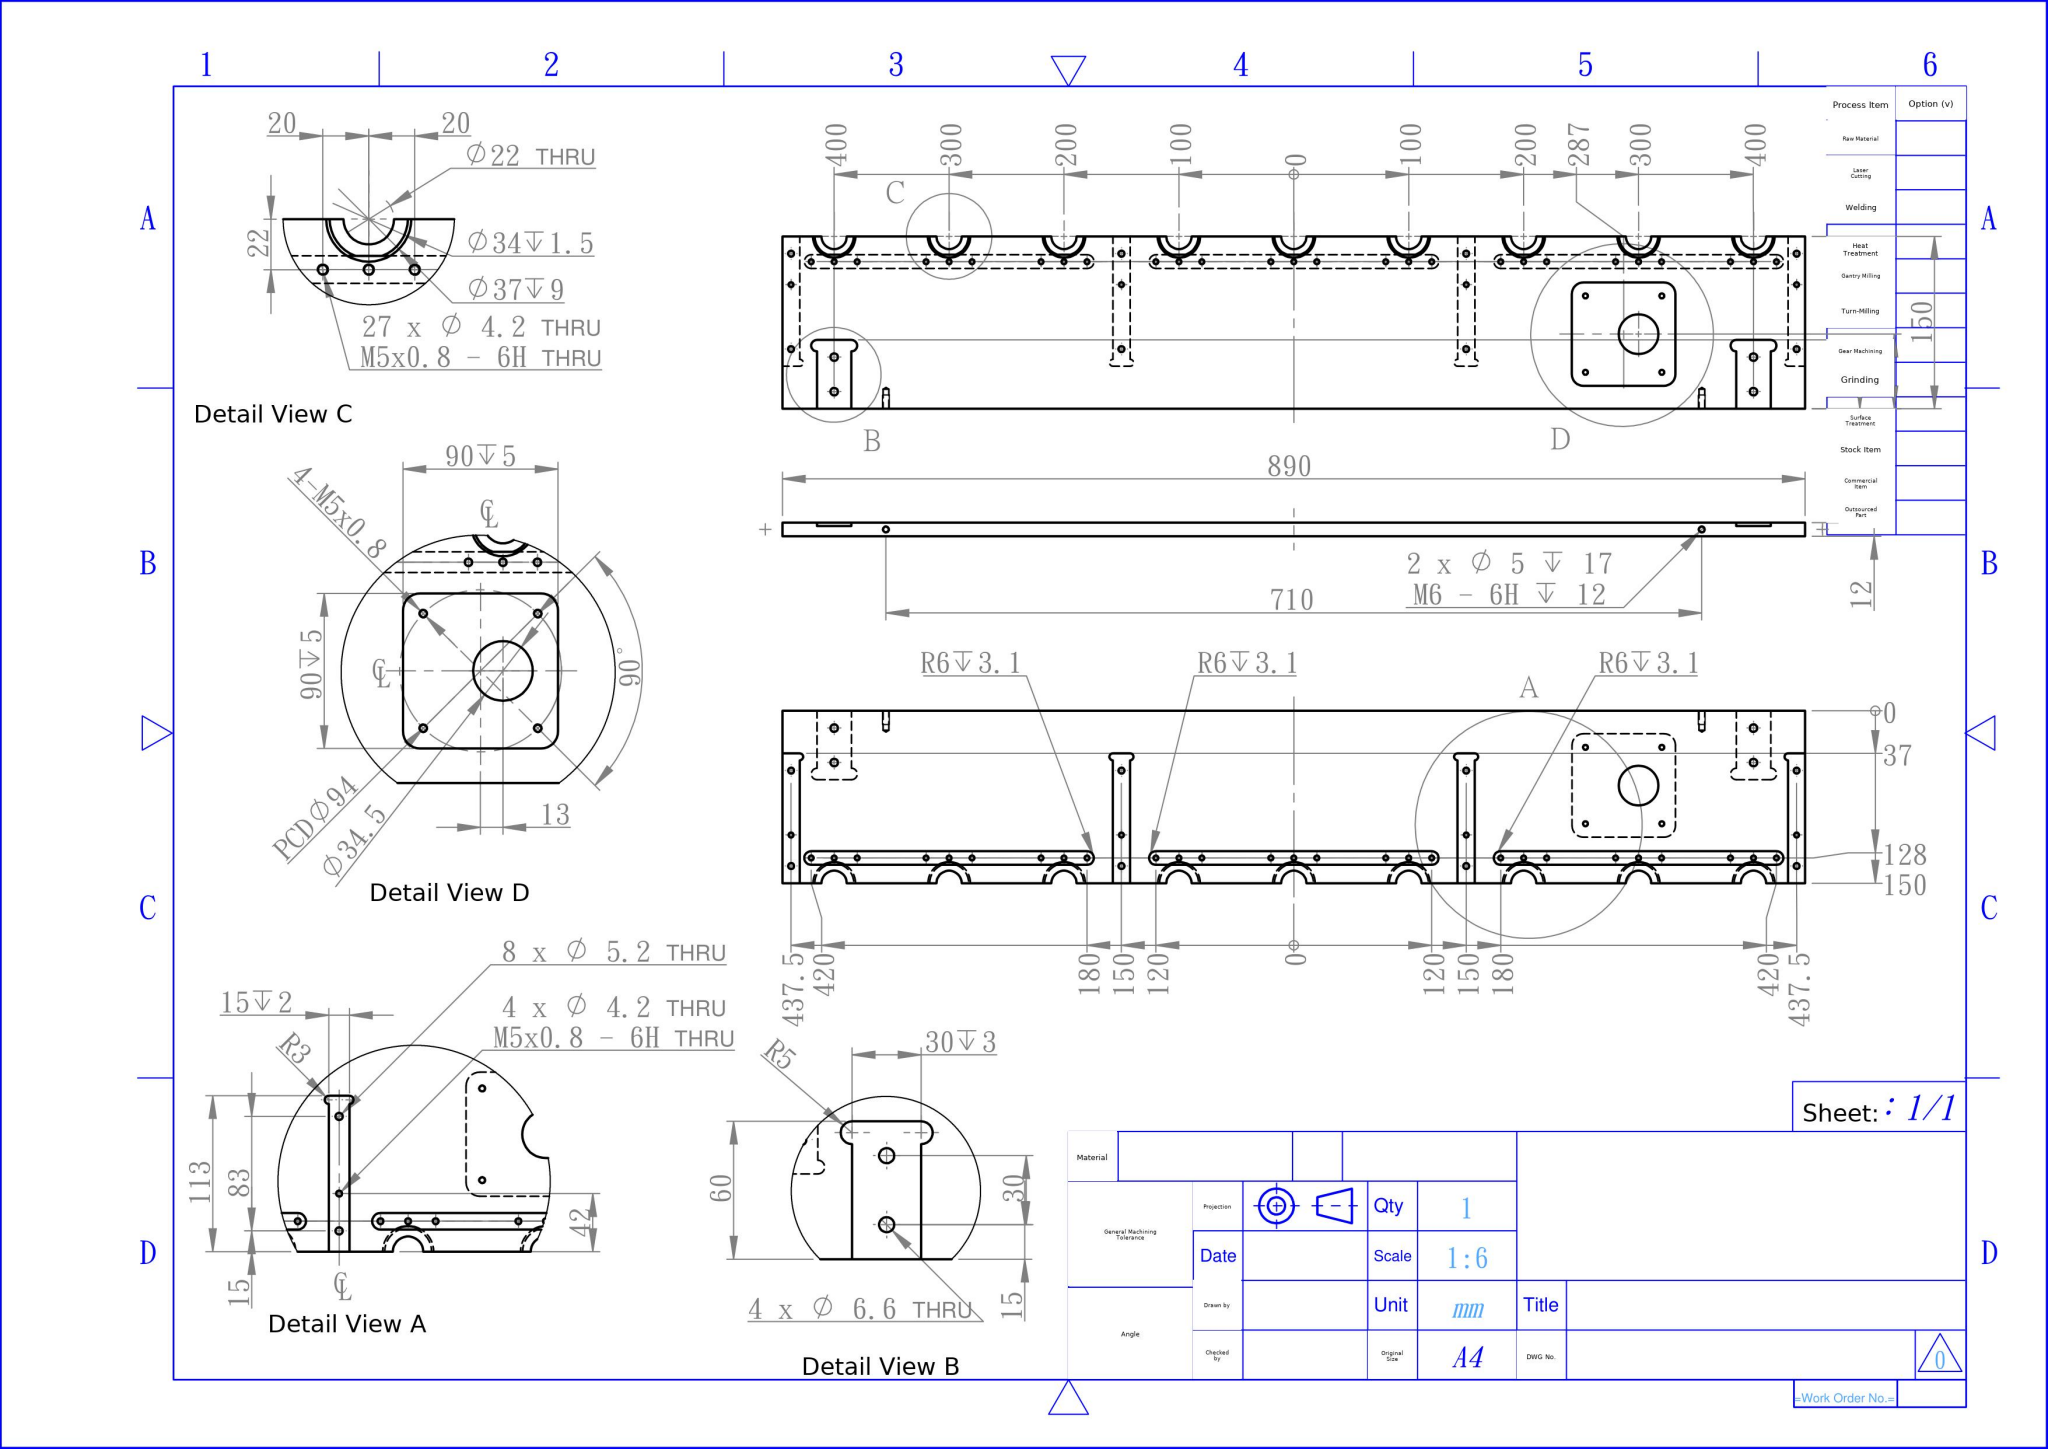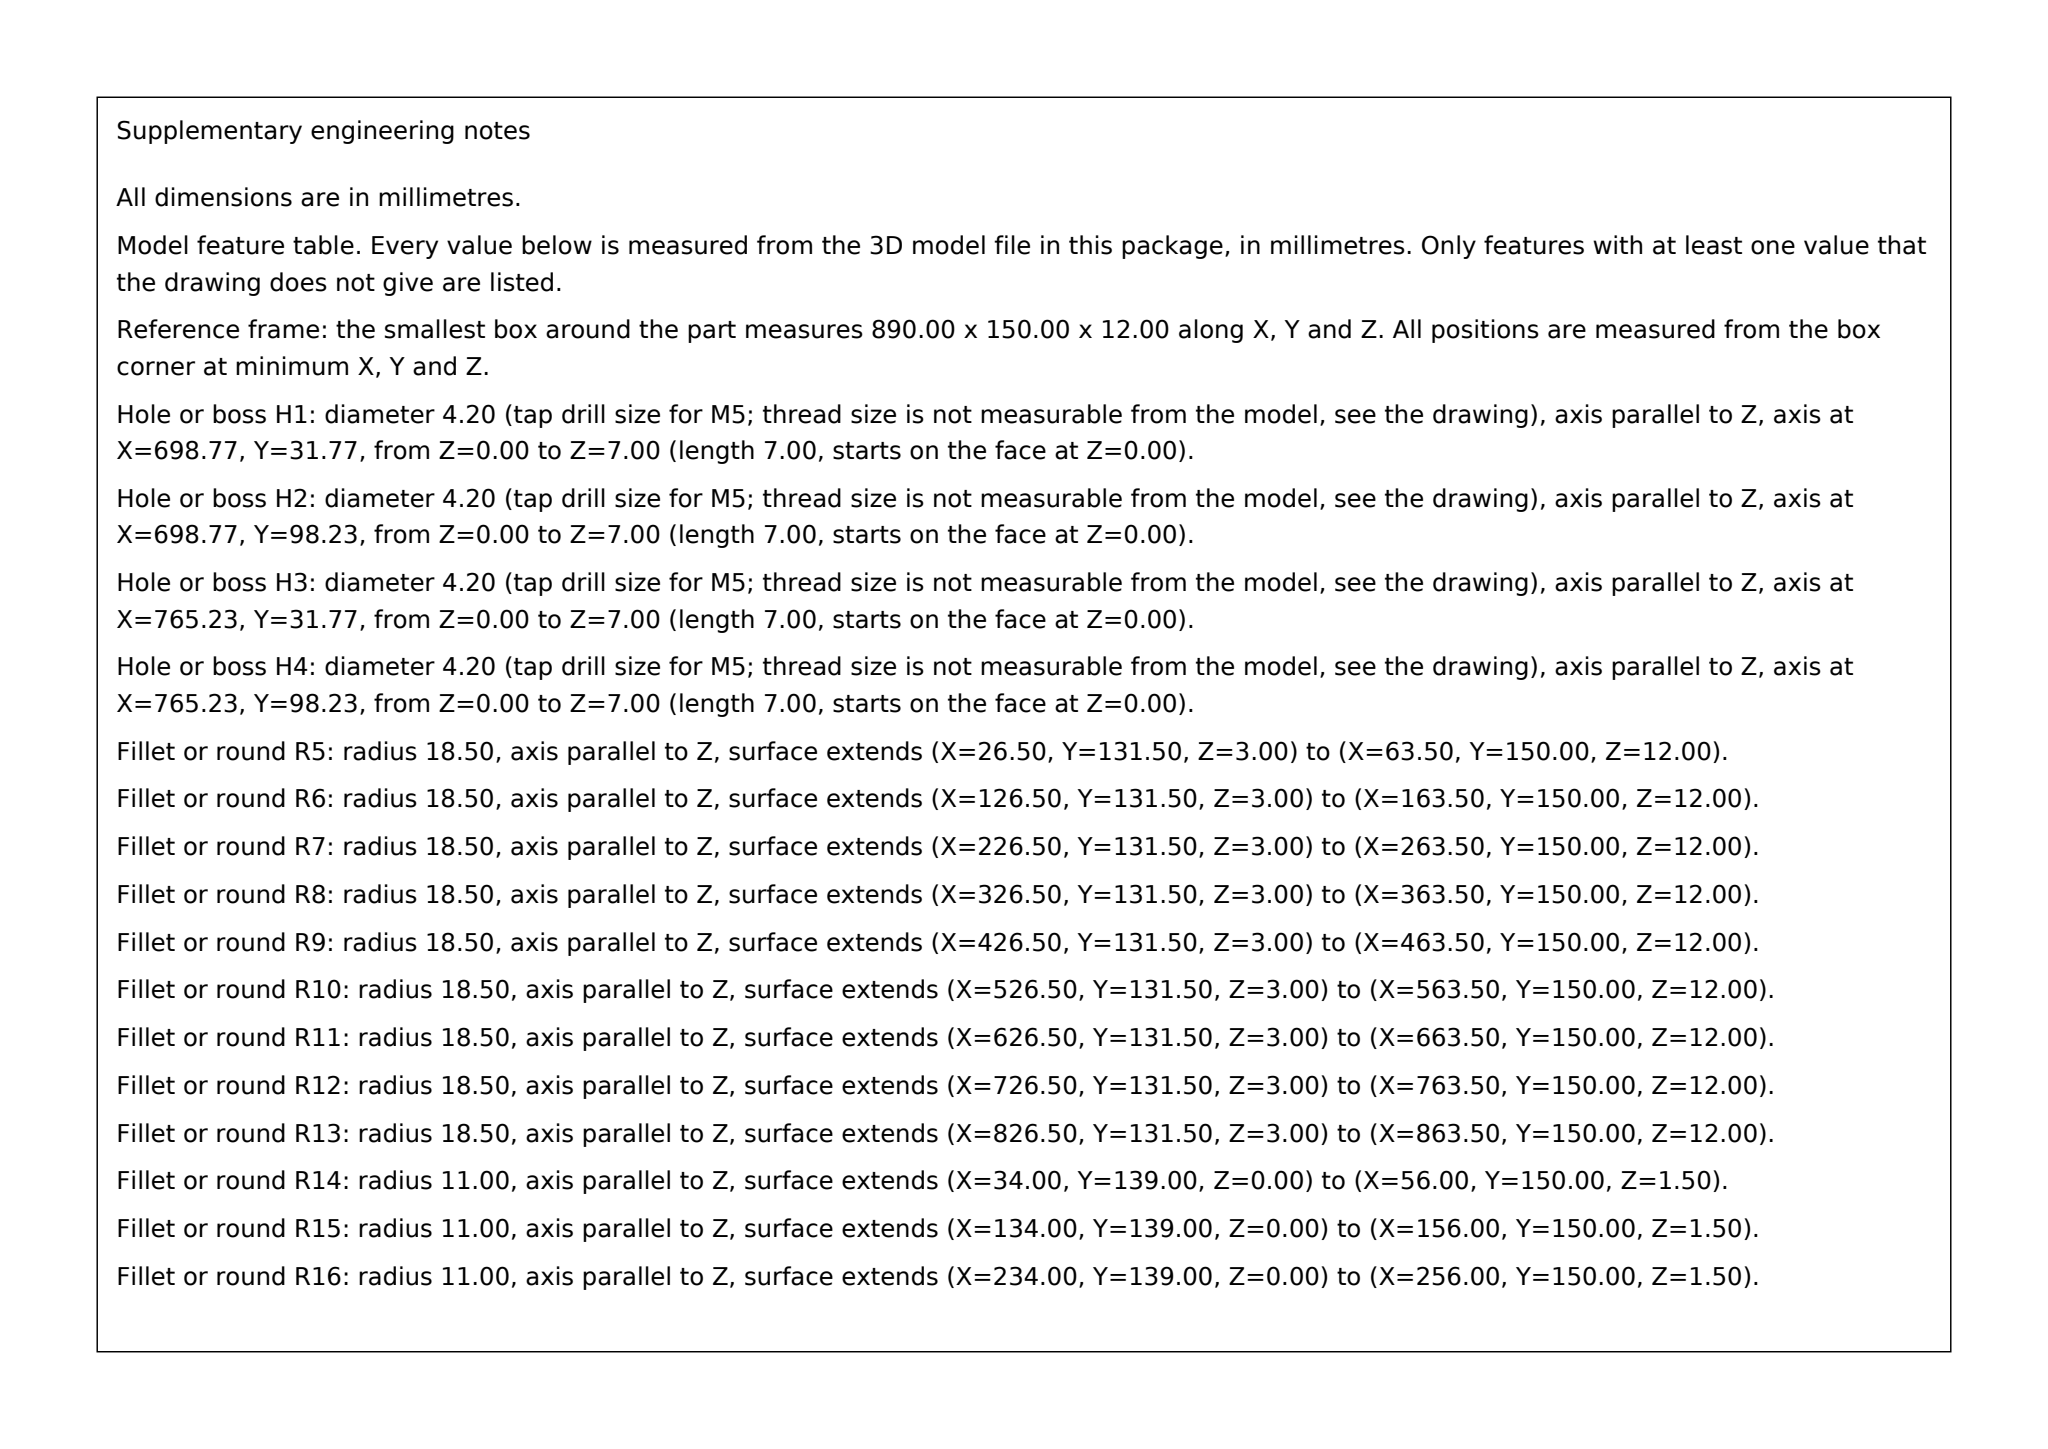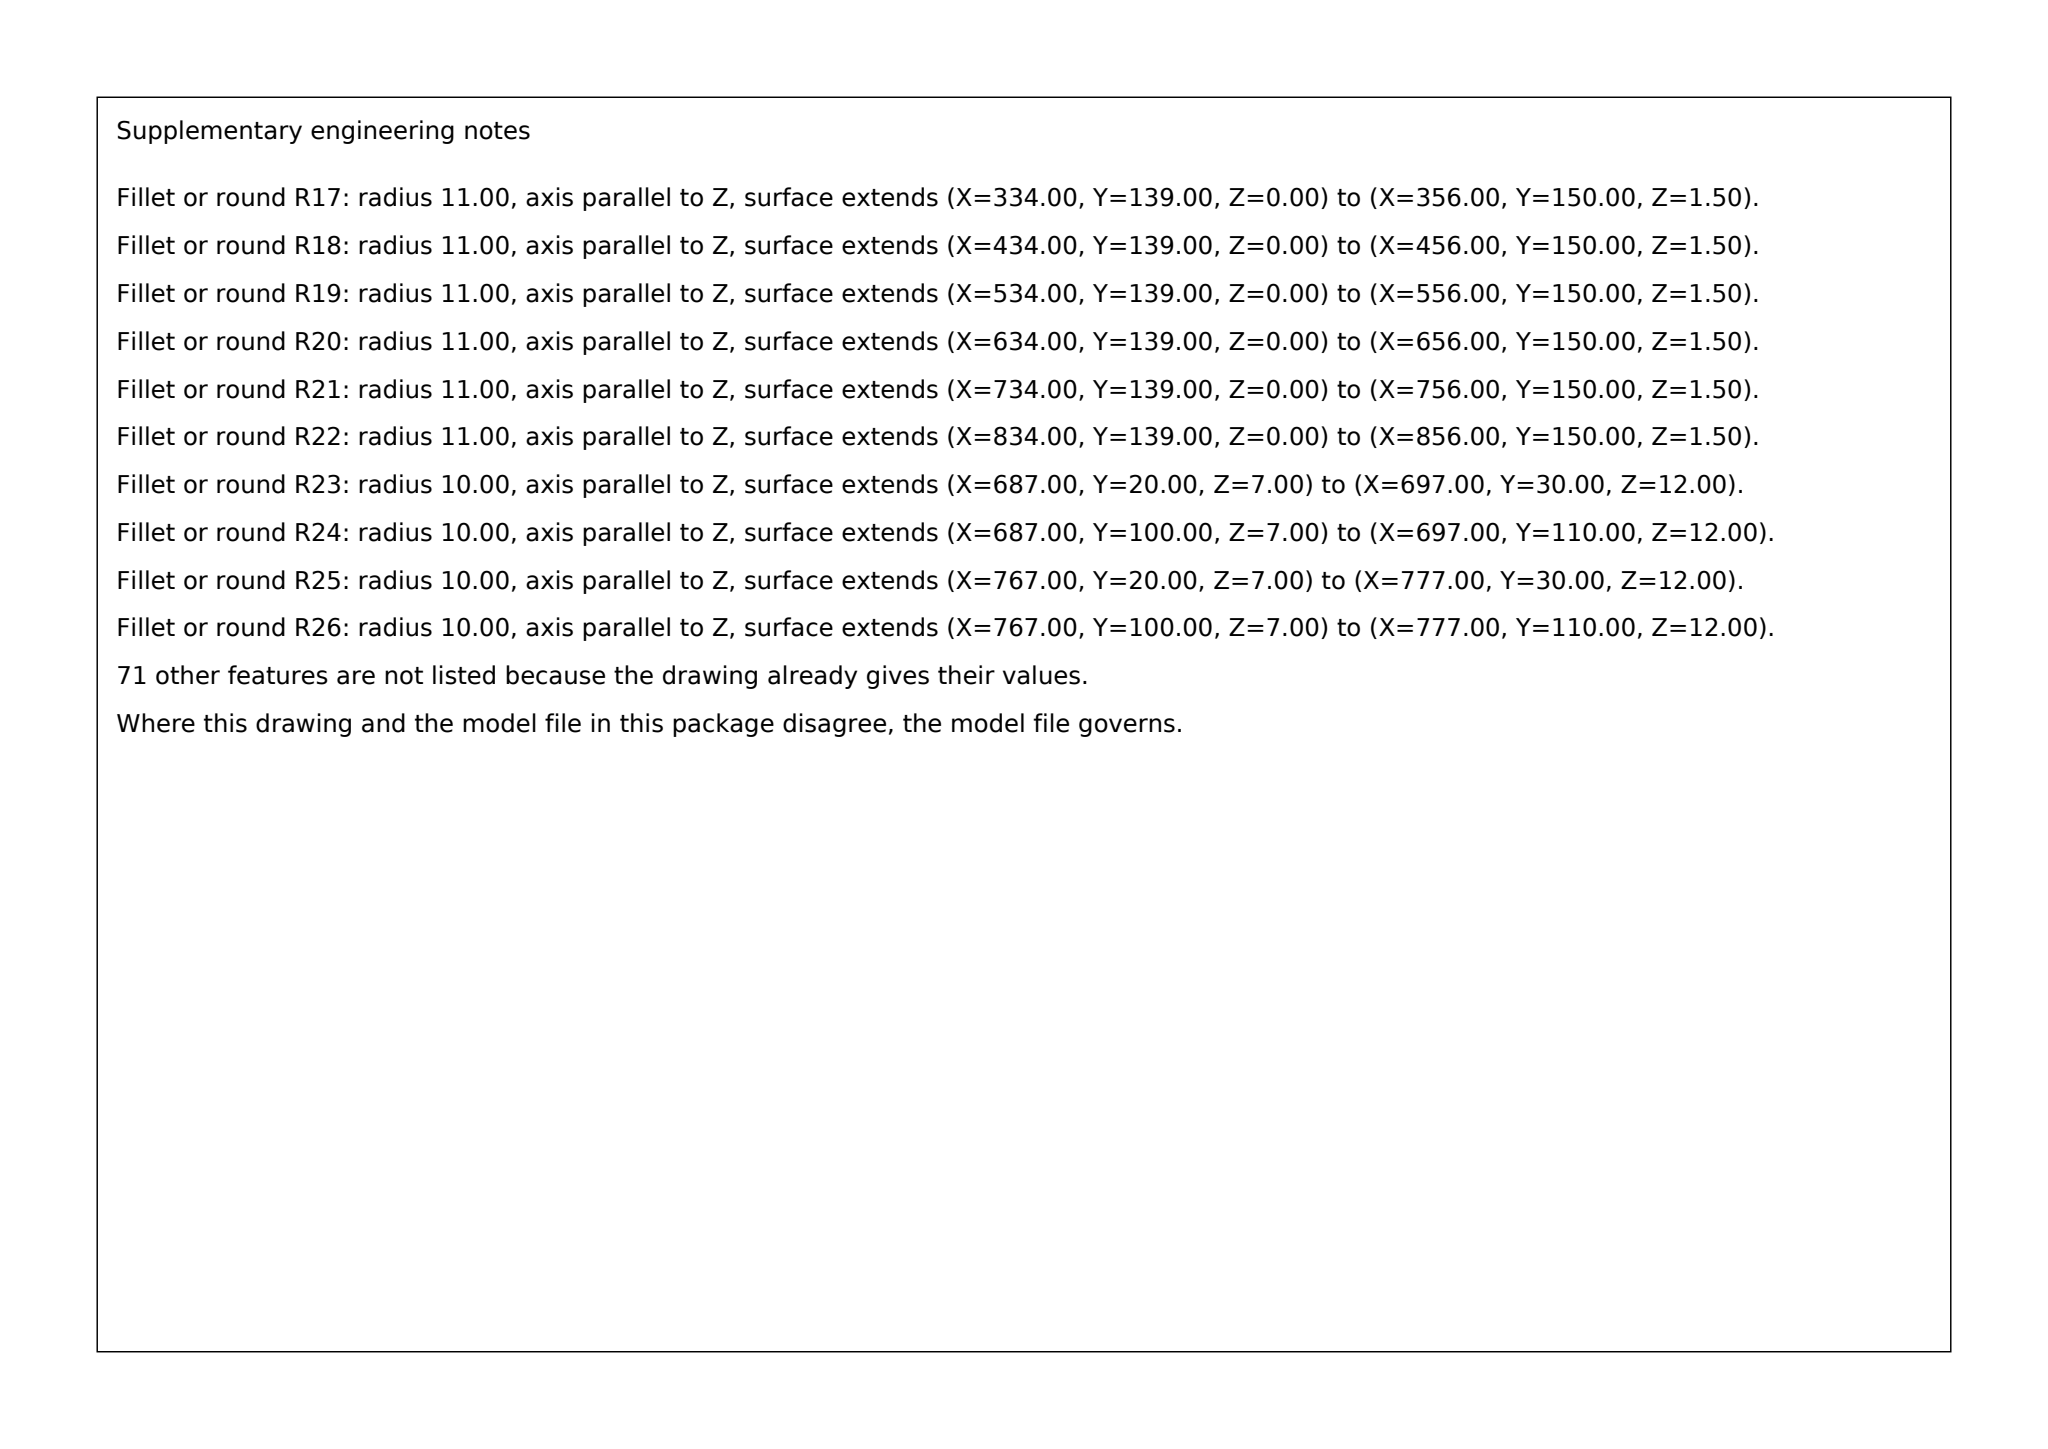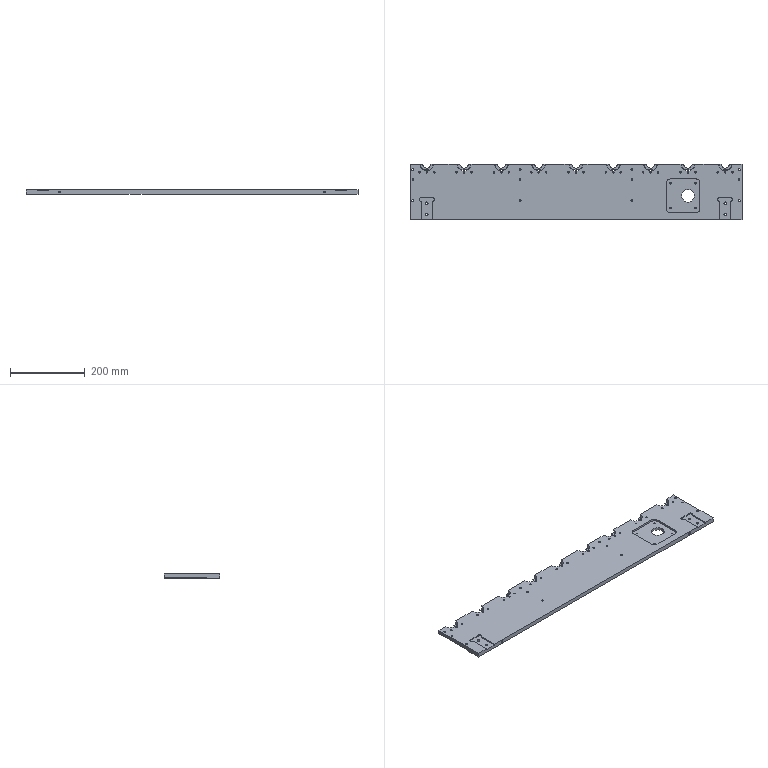Part | SolidWorks | mm | 1 solid | 246 faces | box 890 x 150 x 12 mm | volume 1442552 mm3 | cylinder 164 | plane 78 | cone 4 | commonest cylinder face diameters 4.2 x70 34 x18 5.2 x16 12 x9 6 x9 22 x9 37 x9 6.6 x8
build123d program:
from build123d import *

# Parameters (mm, degrees)
SKETCH1_W                  = 890
SKETCH1_H                  = 150
BOSS_EXTRUDE1_DEPTH        = 12
CUT_EXTRUDE1_DEPTH         = 3
F_6_6_6_6_DIAMETER_HOLE1_D = 6.6
CUT_EXTRUDE2_REACH         = 453.435
SKETCH5_R                  = 11
SKETCH6_R                  = 17
CUT_EXTRUDE3_DEPTH         = 10.5
SKETCH7_R                  = 18.5
CUT_EXTRUDE5_DEPTH         = 9
M5X0_8_TAPPED_HOLE1_D      = 4.2
LINEAR_PATTERN1_COUNT      = 9
LINEAR_PATTERN1_PITCH      = 100
CUT_EXTRUDE6_DEPTH         = 2
F_5_2_5_2_DIAMETER_HOLE1_D = 5.2
M5X0_8_TAPPED_HOLE2_D      = 4.2
CUT_EXTRUDE7_DEPTH         = 3.1
CUT_EXTRUDE8_REACH         = 453.435
SKETCH16_R                 = 17.25
CUT_EXTRUDE9_DEPTH         = 5
M5X0_8_TAPPED_HOLE3_D      = 4.2
M6_TAPPED_HOLE1_D          = 5
M6_TAPPED_HOLE1_DEPTH      = 17
M6_TAPPED_HOLE1_TIP        = 1.502


with BuildPart() as part:
    # Sketch1 → Boss-Extrude1 (new body)
    with BuildSketch(Plane.XY):
        Rectangle(SKETCH1_W, SKETCH1_H)
    extrude(amount=BOSS_EXTRUDE1_DEPTH)

    # Sketch2 → Cut-Extrude1 (cut)
    with BuildSketch(Plane.XY.offset(12)):
        with BuildLine():
            Line((-415, -75), (-415, -25))
            ThreePointArc((-415, -25), (-420, -20), (-415, -15))
            Line((-415, -15), (-385, -15))
            ThreePointArc((-385, -15), (-380, -20), (-385, -25))
            Line((-385, -25), (-385, -75))
            Line((-385, -75), (-415, -75))
        make_face()
        with BuildLine():
            Line((385, -25), (385, -75))
            Line((385, -75), (415, -75))
            Line((415, -75), (415, -25))
            ThreePointArc((415, -25), (420, -20), (415, -15))
            Line((415, -15), (385, -15))
            ThreePointArc((385, -15), (380, -20), (385, -25))
        make_face()
    extrude(amount=-CUT_EXTRUDE1_DEPTH, mode=Mode.SUBTRACT)

    # 6.6 _6.6_ Diameter Hole1 (through all)
    with Locations(Plane.XY.offset(9)):
        with Locations((-400, -30), (-400, -60), (400, -60), (400, -30)):
            Hole(F_6_6_6_6_DIAMETER_HOLE1_D / 2)

    # Sketch5 → Cut-Extrude2 (cut, up to next)
    with BuildSketch(Plane.XY.offset(12), mode=Mode.PRIVATE) as cut_extrude2_sk1:
        with Locations((-400, 75)):
            Circle(SKETCH5_R)
    cut_extrude2_tool1 = extrude(cut_extrude2_sk1.sketch, amount=-CUT_EXTRUDE2_REACH, mode=Mode.PRIVATE) & part.part
    cut_extrude2 = cut_extrude2_tool1.solids().sort_by_distance((-400, 75, 12))[0]
    add(cut_extrude2, mode=Mode.SUBTRACT)

    # Sketch6 → Cut-Extrude3 (cut)
    with BuildSketch(Plane.XY.offset(12)):
        with Locations((-400, 75)):
            Circle(SKETCH6_R)
    cut_extrude3 = extrude(amount=-CUT_EXTRUDE3_DEPTH, mode=Mode.SUBTRACT)

    # Sketch7 → Cut-Extrude5 (cut)
    with BuildSketch(Plane.XY.offset(12)):
        with Locations((-400, 75)):
            Circle(SKETCH7_R)
    cut_extrude5 = extrude(amount=-CUT_EXTRUDE5_DEPTH, mode=Mode.SUBTRACT)

    # M5x0.8 Tapped Hole1 (through all)
    with Locations(Plane.XY.offset(12)):
        with Locations((-420, 53), (-400, 53), (-380, 53)):
            m5x0_8_tapped_hole1 = Hole(M5X0_8_TAPPED_HOLE1_D / 2)

    # Linear Pattern1: Cut-Extrude2, Cut-Extrude3, Cut-Extrude5, M5x0.8 Tapped Hole1 ×9
    with Locations(*[(i * LINEAR_PATTERN1_PITCH, 0, 0) for i in range(1, LINEAR_PATTERN1_COUNT)]):
        add(cut_extrude2, mode=Mode.SUBTRACT)
        add(cut_extrude3, mode=Mode.SUBTRACT)
        add(cut_extrude5, mode=Mode.SUBTRACT)
        add(m5x0_8_tapped_hole1, mode=Mode.SUBTRACT)

    # Sketch10 → Cut-Extrude6 (cut)
    with BuildSketch(Plane(origin=(0, 0, 0), x_dir=(-1, 0, 0), z_dir=(0, 0, -1))):
        with BuildLine():
            Line((445, 75), (430, 75))
            Line((430, 75), (430, -32))
            ThreePointArc((430, -32), (427, -35), (430, -38))
            Line((430, -38), (445, -38))
            ThreePointArc((445, -38), (448, -35), (445, -32))
            Line((445, -32), (445, 75))
        make_face()
        with BuildLine():
            Line((-445, 75), (-430, 75))
            Line((-430, 75), (-430, -32))
            ThreePointArc((-430, -32), (-427, -35), (-430, -38))
            Line((-430, -38), (-445, -38))
            ThreePointArc((-445, -38), (-448, -35), (-445, -32))
            Line((-445, -32), (-445, 75))
        make_face()
        with BuildLine():
            Line((-157.5, 75), (-142.5, 75))
            Line((-142.5, 75), (-142.5, -32))
            ThreePointArc((-142.5, -32), (-139.5, -35), (-142.5, -38))
            Line((-142.5, -38), (-157.5, -38))
            ThreePointArc((-157.5, -38), (-160.5, -35), (-157.5, -32))
            Line((-157.5, -32), (-157.5, 75))
        make_face()
        with BuildLine():
            Line((142.5, 75), (157.5, 75))
            Line((157.5, 75), (157.5, -32))
            ThreePointArc((157.5, -32), (160.5, -35), (157.5, -38))
            Line((157.5, -38), (142.5, -38))
            ThreePointArc((142.5, -38), (139.5, -35), (142.5, -32))
            Line((142.5, -32), (142.5, 75))
        make_face()
    extrude(amount=-CUT_EXTRUDE6_DEPTH, mode=Mode.SUBTRACT)

    # 5.2 _5.2_ Diameter Hole1 (through all)
    with Locations(Plane(origin=(0, 0, 2), x_dir=(-1, 0, 0), z_dir=(0, 0, -1))):
        with Locations((437.5, -23), (437.5, 60), (-437.5, 60), (-437.5, -23), (-150, 60), (-150, -23), (150, 60), (150, -23)):
            Hole(F_5_2_5_2_DIAMETER_HOLE1_D / 2)

    # M5x0.8 Tapped Hole2 (through all)
    with Locations(Plane(origin=(0, 0, 2), x_dir=(-1, 0, 0), z_dir=(0, 0, -1))):
        with Locations((437.5, 33), (150, 33), (-150, 33), (-437.5, 33)):
            Hole(M5X0_8_TAPPED_HOLE2_D / 2)

    # Sketch15 → Cut-Extrude7 (cut)
    with BuildSketch(Plane(origin=(0, 0, 0), x_dir=(-1, 0, 0), z_dir=(0, 0, -1))):
        with BuildLine():
            Line((-420, 59), (-180, 59))
            ThreePointArc((-180, 59), (-174, 53), (-180, 47))
            Line((-180, 47), (-420, 47))
            ThreePointArc((-420, 47), (-426, 53), (-420, 59))
        make_face()
        with BuildLine():
            Line((-120, 59), (120, 59))
            ThreePointArc((120, 59), (126, 53), (120, 47))
            Line((120, 47), (-120, 47))
            ThreePointArc((-120, 47), (-126, 53), (-120, 59))
        make_face()
        with BuildLine():
            Line((180, 59), (420, 59))
            ThreePointArc((420, 59), (426, 53), (420, 47))
            Line((420, 47), (180, 47))
            ThreePointArc((180, 47), (174, 53), (180, 59))
        make_face()
    extrude(amount=-CUT_EXTRUDE7_DEPTH, mode=Mode.SUBTRACT)

    # Sketch16 → Cut-Extrude8 (cut, up to next)
    with BuildSketch(Plane.XY.offset(12), mode=Mode.PRIVATE) as cut_extrude8_sk1:
        with Locations((300, -10)):
            Circle(SKETCH16_R)
    cut_extrude8_tool1 = extrude(cut_extrude8_sk1.sketch, amount=-CUT_EXTRUDE8_REACH, mode=Mode.PRIVATE) & part.part
    add(cut_extrude8_tool1.solids().sort_by_distance((300, -10, 12))[0], mode=Mode.SUBTRACT)

    # Sketch17 → Cut-Extrude9 (cut)
    with BuildSketch(Plane.XY.offset(12)):
        with BuildLine():
            Line((252, 35), (322, 35))
            ThreePointArc((322, 35), (329.071, 32.071), (332, 25))
            Line((332, 25), (332, -45))
            ThreePointArc((332, -45), (329.071, -52.071), (322, -55))
            Line((322, -55), (252, -55))
            ThreePointArc((252, -55), (244.929, -52.071), (242, -45))
            Line((242, -45), (242, 25))
            ThreePointArc((242, 25), (244.929, 32.071), (252, 35))
        make_face()
    extrude(amount=-CUT_EXTRUDE9_DEPTH, mode=Mode.SUBTRACT)

    # M5x0.8 Tapped Hole3 (through all)
    with Locations(Plane.XY.offset(7)):
        with Locations((253.766, -43.234), (253.766, 23.234), (320.234, 23.234), (320.234, -43.234)):
            Hole(M5X0_8_TAPPED_HOLE3_D / 2)

    # M6 Tapped Hole1
    with Locations(Plane(origin=(0, -75, 0), x_dir=(-1, 0, 0), z_dir=(0, -1, 0))):
        with Locations((355, -6), (-355, -6)):
            Hole(M6_TAPPED_HOLE1_D / 2, depth=M6_TAPPED_HOLE1_DEPTH)
            with Locations((0, 0, -(M6_TAPPED_HOLE1_DEPTH + M6_TAPPED_HOLE1_TIP / 2))):  # 118° drill point
                Cone(0, M6_TAPPED_HOLE1_D / 2, M6_TAPPED_HOLE1_TIP, mode=Mode.SUBTRACT)


solid = part.part